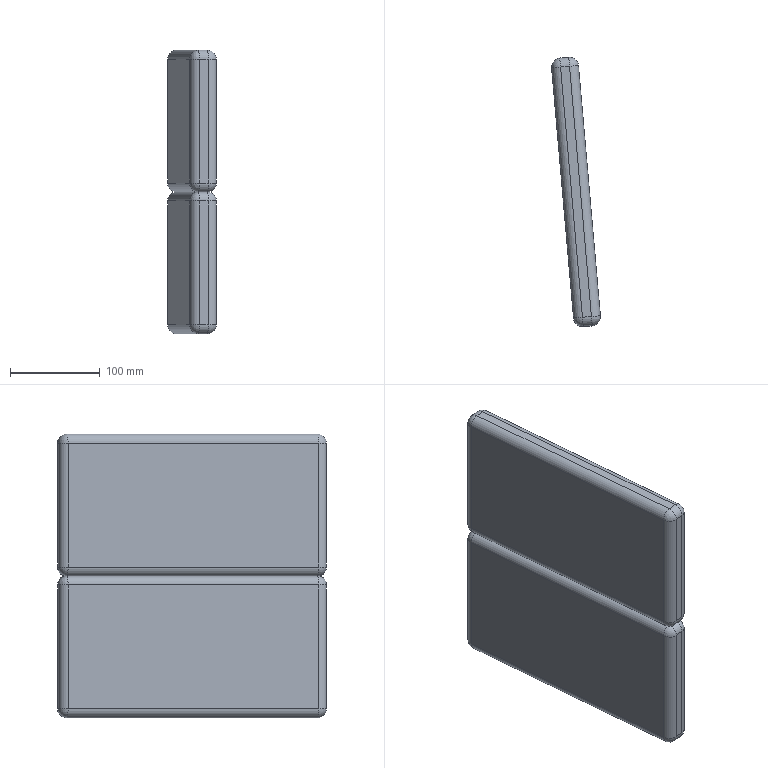Component | SolidWorks | RehabilitationChair-18-2-1 | 1 solid | 50 faces | volume 2764276 mm3 | cylinder 24 | sphere 16 | plane 10 | commonest cylinder face diameters 20 x24